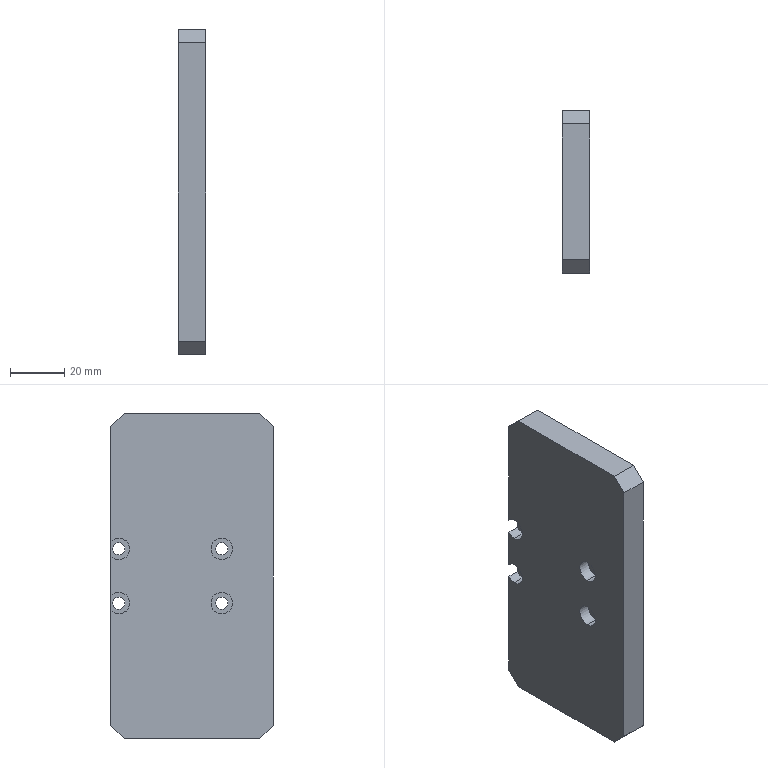Component | SolidWorks | MainRotatingPlate-1 | 1 solid | 32 faces | box 10.01 x 60 x 120 mm | volume 70291 mm3 | cylinder 18 | plane 14 | commonest cylinder face diameters 8 x10 4.5 x8
build123d program:
from build123d import *

# Parameters (mm, degrees)
SKETCH1_W                                       = 120
SKETCH1_H                                       = 60
BOSS_EXTRUDE1_DEPTH                             = 10
CHAMFER1_SIZE                                   = 5
M4_HEX_SOCKET_HEAD_CAP_SCREW_CBORE1_D           = 4.5
M4_HEX_SOCKET_HEAD_CAP_SCREW_CBORE1_DEPTH       = 12.4
M4_HEX_SOCKET_HEAD_CAP_SCREW_CBORE1_CBORE_D     = 8
M4_HEX_SOCKET_HEAD_CAP_SCREW_CBORE1_CBORE_DEPTH = 4.4
M4_HEX_SOCKET_HEAD_CAP_SCREW_CBORE1_TIP         = 1.352


with BuildPart() as part:
    # Sketch1 → Boss-Extrude1 (new body)
    with BuildSketch(Plane.XY):
        Rectangle(SKETCH1_W, SKETCH1_H)
    extrude(amount=BOSS_EXTRUDE1_DEPTH)

    # Chamfer1
    chamfer1_edges = [part.edges().sort_by_distance(p)[0] for p in [
        (-60, 30, 5),
        (60, 30, 5),
        (60, -30, 5),
        (-60, -30, 5),
    ]]
    chamfer(chamfer1_edges, length=CHAMFER1_SIZE)

    # M4 Hex Socket Head Cap Screw CBORE1
    with Locations(Plane.XY.offset(10)):
        with Locations((-10, 11), (10, 11), (-10, -27), (10, -27)):
            CounterBoreHole(M4_HEX_SOCKET_HEAD_CAP_SCREW_CBORE1_D / 2, M4_HEX_SOCKET_HEAD_CAP_SCREW_CBORE1_CBORE_D / 2, M4_HEX_SOCKET_HEAD_CAP_SCREW_CBORE1_CBORE_DEPTH, depth=M4_HEX_SOCKET_HEAD_CAP_SCREW_CBORE1_DEPTH)
            with Locations((0, 0, -(M4_HEX_SOCKET_HEAD_CAP_SCREW_CBORE1_DEPTH + M4_HEX_SOCKET_HEAD_CAP_SCREW_CBORE1_TIP / 2))):  # 118° drill point
                Cone(0, M4_HEX_SOCKET_HEAD_CAP_SCREW_CBORE1_D / 2, M4_HEX_SOCKET_HEAD_CAP_SCREW_CBORE1_TIP, mode=Mode.SUBTRACT)


solid = part.part

# Placed as in the assembly
solid = solid.moved(Location((1842.163, 3833.741, 1079.241), (180, -90, 0)))
STEP:
#1=COLOUR_RGB('',0.7922,0.8196,0.9333);
#2=FILL_AREA_STYLE_COLOUR('',#1);
#3=FILL_AREA_STYLE('',(#2));
#4=SURFACE_STYLE_FILL_AREA(#3);
#5=SURFACE_SIDE_STYLE('',(#4));
#6=SURFACE_STYLE_USAGE(.BOTH.,#5);
#7=PRESENTATION_STYLE_ASSIGNMENT((#6));
#8=CARTESIAN_POINT('',(72.306,150.502,43.041));
#9=VERTEX_POINT('',#8);
#10=CARTESIAN_POINT('',(72.306,150.502,42.726));
#11=VERTEX_POINT('',#10);
#12=CARTESIAN_POINT('',(72.306,150.502,42.884));
#13=DIRECTION('',(-1.,-0.0001552,-0.));
#14=DIRECTION('',(0.,0.,-1.));
#15=AXIS2_PLACEMENT_3D('',#12,#13,#14);
#16=CIRCLE('',#15,0.1575);
#17=EDGE_CURVE('',#9,#11,#16,.T.);
#18=ORIENTED_EDGE('',*,*,#17,.F.);
#19=CARTESIAN_POINT('',(72.132,150.502,43.041));
#20=VERTEX_POINT('',#19);
#21=CARTESIAN_POINT('',(72.132,150.502,43.041));
#22=DIRECTION('',(-1.,-0.0001552,-0.));
#23=VECTOR('',#22,39.37);
#24=LINE('',#21,#23);
#25=EDGE_CURVE('',#9,#20,#24,.T.);
#26=ORIENTED_EDGE('',*,*,#25,.T.);
#27=CARTESIAN_POINT('',(72.132,150.502,42.726));
#28=VERTEX_POINT('',#27);
#29=CARTESIAN_POINT('',(72.132,150.502,42.884));
#30=DIRECTION('',(-1.,-0.0001552,-0.));
#31=DIRECTION('',(0.,0.,-1.));
#32=AXIS2_PLACEMENT_3D('',#29,#30,#31);
#33=CIRCLE('',#32,0.1575);
#34=EDGE_CURVE('',#20,#28,#33,.T.);
#35=ORIENTED_EDGE('',*,*,#34,.T.);
#36=CARTESIAN_POINT('',(72.132,150.502,42.726));
#37=DIRECTION('',(-1.,-0.0001552,-0.));
#38=VECTOR('',#37,39.37);
#39=LINE('',#36,#38);
#40=EDGE_CURVE('',#11,#28,#39,.T.);
#41=ORIENTED_EDGE('',*,*,#40,.F.);
#42=EDGE_LOOP('',(#18,#26,#35,#41));
#43=FACE_OUTER_BOUND('',#42,.T.);
#44=CARTESIAN_POINT('',(72.132,150.502,42.884));
#45=DIRECTION('',(-1.,-0.0001552,-0.));
#46=DIRECTION('',(0.,0.,-1.));
#47=AXIS2_PLACEMENT_3D('',#44,#45,#46);
#48=CYLINDRICAL_SURFACE('',#47,0.1575);
#49=ADVANCED_FACE('',(#43),#48,.F.);
#50=CARTESIAN_POINT('',(72.526,150.502,42.972));
#51=VERTEX_POINT('',#50);
#52=CARTESIAN_POINT('',(72.526,150.502,42.795));
#53=VERTEX_POINT('',#52);
#54=CARTESIAN_POINT('',(72.526,150.502,42.884));
#55=DIRECTION('',(-1.,-0.0001552,-0.));
#56=DIRECTION('',(0.,0.,-1.));
#57=AXIS2_PLACEMENT_3D('',#54,#55,#56);
#58=CIRCLE('',#57,0.08858);
#59=EDGE_CURVE('',#51,#53,#58,.T.);
#60=ORIENTED_EDGE('',*,*,#59,.F.);
#61=CARTESIAN_POINT('',(72.306,150.502,42.972));
#62=VERTEX_POINT('',#61);
#63=CARTESIAN_POINT('',(72.132,150.502,42.972));
#64=DIRECTION('',(-1.,-0.0001552,-0.));
#65=VECTOR('',#64,39.37);
#66=LINE('',#63,#65);
#67=EDGE_CURVE('',#51,#62,#66,.T.);
#68=ORIENTED_EDGE('',*,*,#67,.T.);
#69=CARTESIAN_POINT('',(72.306,150.502,42.795));
#70=VERTEX_POINT('',#69);
#71=CARTESIAN_POINT('',(72.306,150.502,42.884));
#72=DIRECTION('',(-1.,-0.0001552,-0.));
#73=DIRECTION('',(0.,0.,-1.));
#74=AXIS2_PLACEMENT_3D('',#71,#72,#73);
#75=CIRCLE('',#74,0.08858);
#76=EDGE_CURVE('',#62,#70,#75,.T.);
#77=ORIENTED_EDGE('',*,*,#76,.T.);
#78=CARTESIAN_POINT('',(72.132,150.502,42.795));
#79=DIRECTION('',(-1.,-0.0001552,-0.));
#80=VECTOR('',#79,39.37);
#81=LINE('',#78,#80);
#82=EDGE_CURVE('',#53,#70,#81,.T.);
#83=ORIENTED_EDGE('',*,*,#82,.F.);
#84=EDGE_LOOP('',(#60,#68,#77,#83));
#85=FACE_OUTER_BOUND('',#84,.T.);
#86=CARTESIAN_POINT('',(72.132,150.502,42.884));
#87=DIRECTION('',(-1.,-0.0001552,-0.));
#88=DIRECTION('',(0.,0.,-1.));
#89=AXIS2_PLACEMENT_3D('',#86,#87,#88);
#90=CYLINDRICAL_SURFACE('',#89,0.08858);
#91=ADVANCED_FACE('',(#85),#90,.F.);
#92=CARTESIAN_POINT('',(72.306,150.502,42.254));
#93=VERTEX_POINT('',#92);
#94=CARTESIAN_POINT('',(72.306,150.502,41.939));
#95=VERTEX_POINT('',#94);
#96=CARTESIAN_POINT('',(72.306,150.502,42.096));
#97=DIRECTION('',(-1.,-0.0001552,-0.));
#98=DIRECTION('',(0.,0.,-1.));
#99=AXIS2_PLACEMENT_3D('',#96,#97,#98);
#100=CIRCLE('',#99,0.1575);
#101=EDGE_CURVE('',#93,#95,#100,.T.);
#102=ORIENTED_EDGE('',*,*,#101,.F.);
#103=CARTESIAN_POINT('',(72.132,150.502,42.254));
#104=VERTEX_POINT('',#103);
#105=CARTESIAN_POINT('',(72.132,150.502,42.254));
#106=DIRECTION('',(-1.,-0.0001552,-0.));
#107=VECTOR('',#106,39.37);
#108=LINE('',#105,#107);
#109=EDGE_CURVE('',#93,#104,#108,.T.);
#110=ORIENTED_EDGE('',*,*,#109,.T.);
#111=CARTESIAN_POINT('',(72.132,150.502,41.939));
#112=VERTEX_POINT('',#111);
#113=CARTESIAN_POINT('',(72.132,150.502,42.096));
#114=DIRECTION('',(-1.,-0.0001552,-0.));
#115=DIRECTION('',(0.,0.,-1.));
#116=AXIS2_PLACEMENT_3D('',#113,#114,#115);
#117=CIRCLE('',#116,0.1575);
#118=EDGE_CURVE('',#104,#112,#117,.T.);
#119=ORIENTED_EDGE('',*,*,#118,.T.);
#120=CARTESIAN_POINT('',(72.132,150.502,41.939));
#121=DIRECTION('',(-1.,-0.0001552,-0.));
#122=VECTOR('',#121,39.37);
#123=LINE('',#120,#122);
#124=EDGE_CURVE('',#95,#112,#123,.T.);
#125=ORIENTED_EDGE('',*,*,#124,.F.);
#126=EDGE_LOOP('',(#102,#110,#119,#125));
#127=FACE_OUTER_BOUND('',#126,.T.);
#128=CARTESIAN_POINT('',(72.132,150.502,42.096));
#129=DIRECTION('',(-1.,-0.0001552,-0.));
#130=DIRECTION('',(0.,0.,-1.));
#131=AXIS2_PLACEMENT_3D('',#128,#129,#130);
#132=CYLINDRICAL_SURFACE('',#131,0.1575);
#133=ADVANCED_FACE('',(#127),#132,.F.);
#134=CARTESIAN_POINT('',(72.526,150.502,42.185));
#135=VERTEX_POINT('',#134);
#136=CARTESIAN_POINT('',(72.526,150.502,42.008));
#137=VERTEX_POINT('',#136);
#138=CARTESIAN_POINT('',(72.526,150.502,42.096));
#139=DIRECTION('',(-1.,-0.0001552,-0.));
#140=DIRECTION('',(0.,0.,-1.));
#141=AXIS2_PLACEMENT_3D('',#138,#139,#140);
#142=CIRCLE('',#141,0.08858);
#143=EDGE_CURVE('',#135,#137,#142,.T.);
#144=ORIENTED_EDGE('',*,*,#143,.F.);
#145=CARTESIAN_POINT('',(72.306,150.502,42.185));
#146=VERTEX_POINT('',#145);
#147=CARTESIAN_POINT('',(72.132,150.502,42.185));
#148=DIRECTION('',(-1.,-0.0001552,-0.));
#149=VECTOR('',#148,39.37);
#150=LINE('',#147,#149);
#151=EDGE_CURVE('',#135,#146,#150,.T.);
#152=ORIENTED_EDGE('',*,*,#151,.T.);
#153=CARTESIAN_POINT('',(72.306,150.502,42.008));
#154=VERTEX_POINT('',#153);
#155=CARTESIAN_POINT('',(72.306,150.502,42.096));
#156=DIRECTION('',(-1.,-0.0001552,-0.));
#157=DIRECTION('',(0.,0.,-1.));
#158=AXIS2_PLACEMENT_3D('',#155,#156,#157);
#159=CIRCLE('',#158,0.08858);
#160=EDGE_CURVE('',#146,#154,#159,.T.);
#161=ORIENTED_EDGE('',*,*,#160,.T.);
#162=CARTESIAN_POINT('',(72.132,150.502,42.008));
#163=DIRECTION('',(-1.,-0.0001552,-0.));
#164=VECTOR('',#163,39.37);
#165=LINE('',#162,#164);
#166=EDGE_CURVE('',#137,#154,#165,.T.);
#167=ORIENTED_EDGE('',*,*,#166,.F.);
#168=EDGE_LOOP('',(#144,#152,#161,#167));
#169=FACE_OUTER_BOUND('',#168,.T.);
#170=CARTESIAN_POINT('',(72.132,150.502,42.096));
#171=DIRECTION('',(-1.,-0.0001552,-0.));
#172=DIRECTION('',(0.,0.,-1.));
#173=AXIS2_PLACEMENT_3D('',#170,#171,#172);
#174=CYLINDRICAL_SURFACE('',#173,0.08858);
#175=ADVANCED_FACE('',(#169),#174,.F.);
#176=CARTESIAN_POINT('',(72.526,151.998,42.972));
#177=VERTEX_POINT('',#176);
#178=CARTESIAN_POINT('',(72.526,151.998,42.795));
#179=VERTEX_POINT('',#178);
#180=CARTESIAN_POINT('',(72.526,151.998,42.884));
#181=DIRECTION('',(-1.,-0.0001552,-0.));
#182=DIRECTION('',(0.,0.,-1.));
#183=AXIS2_PLACEMENT_3D('',#180,#181,#182);
#184=CIRCLE('',#183,0.08858);
#185=EDGE_CURVE('',#177,#179,#184,.T.);
#186=ORIENTED_EDGE('',*,*,#185,.F.);
#187=CARTESIAN_POINT('',(72.305,151.998,42.972));
#188=VERTEX_POINT('',#187);
#189=CARTESIAN_POINT('',(72.132,151.998,42.972));
#190=DIRECTION('',(-1.,-0.0001552,-0.));
#191=VECTOR('',#190,39.37);
#192=LINE('',#189,#191);
#193=EDGE_CURVE('',#177,#188,#192,.T.);
#194=ORIENTED_EDGE('',*,*,#193,.T.);
#195=CARTESIAN_POINT('',(72.305,151.998,42.795));
#196=VERTEX_POINT('',#195);
#197=CARTESIAN_POINT('',(72.305,151.998,42.884));
#198=DIRECTION('',(-1.,-0.0001552,-0.));
#199=DIRECTION('',(0.,0.,-1.));
#200=AXIS2_PLACEMENT_3D('',#197,#198,#199);
#201=CIRCLE('',#200,0.08858);
#202=EDGE_CURVE('',#188,#196,#201,.T.);
#203=ORIENTED_EDGE('',*,*,#202,.T.);
#204=CARTESIAN_POINT('',(72.132,151.998,42.795));
#205=DIRECTION('',(-1.,-0.0001552,-0.));
#206=VECTOR('',#205,39.37);
#207=LINE('',#204,#206);
#208=EDGE_CURVE('',#179,#196,#207,.T.);
#209=ORIENTED_EDGE('',*,*,#208,.F.);
#210=EDGE_LOOP('',(#186,#194,#203,#209));
#211=FACE_OUTER_BOUND('',#210,.T.);
#212=CARTESIAN_POINT('',(72.132,151.998,42.884));
#213=DIRECTION('',(-1.,-0.0001552,-0.));
#214=DIRECTION('',(0.,0.,-1.));
#215=AXIS2_PLACEMENT_3D('',#212,#213,#214);
#216=CYLINDRICAL_SURFACE('',#215,0.08858);
#217=ADVANCED_FACE('',(#211),#216,.F.);
#218=CARTESIAN_POINT('',(72.305,151.998,43.041));
#219=VERTEX_POINT('',#218);
#220=CARTESIAN_POINT('',(72.305,152.116,42.988));
#221=VERTEX_POINT('',#220);
#222=CARTESIAN_POINT('',(72.305,151.998,42.884));
#223=DIRECTION('',(-1.,-0.0001552,-0.));
#224=DIRECTION('',(0.,0.,-1.));
#225=AXIS2_PLACEMENT_3D('',#222,#223,#224);
#226=CIRCLE('',#225,0.1575);
#227=EDGE_CURVE('',#219,#221,#226,.T.);
#228=ORIENTED_EDGE('',*,*,#227,.F.);
#229=CARTESIAN_POINT('',(72.132,151.998,43.041));
#230=VERTEX_POINT('',#229);
#231=CARTESIAN_POINT('',(72.132,151.998,43.041));
#232=DIRECTION('',(-1.,-0.0001552,-0.));
#233=VECTOR('',#232,39.37);
#234=LINE('',#231,#233);
#235=EDGE_CURVE('',#219,#230,#234,.T.);
#236=ORIENTED_EDGE('',*,*,#235,.T.);
#237=CARTESIAN_POINT('',(72.132,152.116,42.988));
#238=VERTEX_POINT('',#237);
#239=CARTESIAN_POINT('',(72.132,151.998,42.884));
#240=DIRECTION('',(-1.,-0.0001552,-0.));
#241=DIRECTION('',(0.,0.,-1.));
#242=AXIS2_PLACEMENT_3D('',#239,#240,#241);
#243=CIRCLE('',#242,0.1575);
#244=EDGE_CURVE('',#230,#238,#243,.T.);
#245=ORIENTED_EDGE('',*,*,#244,.T.);
#246=CARTESIAN_POINT('',(72.132,152.116,42.988));
#247=DIRECTION('',(-1.,-0.0001552,-0.));
#248=VECTOR('',#247,39.37);
#249=LINE('',#246,#248);
#250=EDGE_CURVE('',#221,#238,#249,.T.);
#251=ORIENTED_EDGE('',*,*,#250,.F.);
#252=EDGE_LOOP('',(#228,#236,#245,#251));
#253=FACE_OUTER_BOUND('',#252,.T.);
#254=CARTESIAN_POINT('',(72.132,151.998,42.884));
#255=DIRECTION('',(-1.,-0.0001552,-0.));
#256=DIRECTION('',(0.,0.,-1.));
#257=AXIS2_PLACEMENT_3D('',#254,#255,#256);
#258=CYLINDRICAL_SURFACE('',#257,0.1575);
#259=ADVANCED_FACE('',(#253),#258,.F.);
#260=ORIENTED_EDGE('',*,*,#235,.F.);
#261=CARTESIAN_POINT('',(72.305,151.998,42.726));
#262=VERTEX_POINT('',#261);
#263=CARTESIAN_POINT('',(72.305,151.998,42.884));
#264=DIRECTION('',(-1.,-0.0001552,-0.));
#265=DIRECTION('',(0.,0.,-1.));
#266=AXIS2_PLACEMENT_3D('',#263,#264,#265);
#267=CIRCLE('',#266,0.1575);
#268=EDGE_CURVE('',#262,#219,#267,.T.);
#269=ORIENTED_EDGE('',*,*,#268,.F.);
#270=CARTESIAN_POINT('',(72.132,151.998,42.726));
#271=VERTEX_POINT('',#270);
#272=CARTESIAN_POINT('',(72.132,151.998,42.726));
#273=DIRECTION('',(-1.,-0.0001552,-0.));
#274=VECTOR('',#273,39.37);
#275=LINE('',#272,#274);
#276=EDGE_CURVE('',#262,#271,#275,.T.);
#277=ORIENTED_EDGE('',*,*,#276,.T.);
#278=CARTESIAN_POINT('',(72.132,151.998,42.884));
#279=DIRECTION('',(-1.,-0.0001552,-0.));
#280=DIRECTION('',(0.,0.,-1.));
#281=AXIS2_PLACEMENT_3D('',#278,#279,#280);
#282=CIRCLE('',#281,0.1575);
#283=EDGE_CURVE('',#271,#230,#282,.T.);
#284=ORIENTED_EDGE('',*,*,#283,.T.);
#285=EDGE_LOOP('',(#260,#269,#277,#284));
#286=FACE_OUTER_BOUND('',#285,.T.);
#287=CARTESIAN_POINT('',(72.132,151.998,42.884));
#288=DIRECTION('',(-1.,-0.0001552,-0.));
#289=DIRECTION('',(0.,0.,-1.));
#290=AXIS2_PLACEMENT_3D('',#287,#288,#289);
#291=CYLINDRICAL_SURFACE('',#290,0.1575);
#292=ADVANCED_FACE('',(#286),#291,.F.);
#293=CARTESIAN_POINT('',(72.526,151.998,42.185));
#294=VERTEX_POINT('',#293);
#295=CARTESIAN_POINT('',(72.526,151.998,42.008));
#296=VERTEX_POINT('',#295);
#297=CARTESIAN_POINT('',(72.526,151.998,42.096));
#298=DIRECTION('',(-1.,-0.0001552,-0.));
#299=DIRECTION('',(0.,0.,-1.));
#300=AXIS2_PLACEMENT_3D('',#297,#298,#299);
#301=CIRCLE('',#300,0.08858);
#302=EDGE_CURVE('',#294,#296,#301,.T.);
#303=ORIENTED_EDGE('',*,*,#302,.F.);
#304=CARTESIAN_POINT('',(72.305,151.998,42.185));
#305=VERTEX_POINT('',#304);
#306=CARTESIAN_POINT('',(72.132,151.998,42.185));
#307=DIRECTION('',(-1.,-0.0001552,-0.));
#308=VECTOR('',#307,39.37);
#309=LINE('',#306,#308);
#310=EDGE_CURVE('',#294,#305,#309,.T.);
#311=ORIENTED_EDGE('',*,*,#310,.T.);
#312=CARTESIAN_POINT('',(72.305,151.998,42.008));
#313=VERTEX_POINT('',#312);
#314=CARTESIAN_POINT('',(72.305,151.998,42.096));
#315=DIRECTION('',(-1.,-0.0001552,-0.));
#316=DIRECTION('',(0.,0.,-1.));
#317=AXIS2_PLACEMENT_3D('',#314,#315,#316);
#318=CIRCLE('',#317,0.08858);
#319=EDGE_CURVE('',#305,#313,#318,.T.);
#320=ORIENTED_EDGE('',*,*,#319,.T.);
#321=CARTESIAN_POINT('',(72.132,151.998,42.008));
#322=DIRECTION('',(-1.,-0.0001552,-0.));
#323=VECTOR('',#322,39.37);
#324=LINE('',#321,#323);
#325=EDGE_CURVE('',#296,#313,#324,.T.);
#326=ORIENTED_EDGE('',*,*,#325,.F.);
#327=EDGE_LOOP('',(#303,#311,#320,#326));
#328=FACE_OUTER_BOUND('',#327,.T.);
#329=CARTESIAN_POINT('',(72.132,151.998,42.096));
#330=DIRECTION('',(-1.,-0.0001552,-0.));
#331=DIRECTION('',(0.,0.,-1.));
#332=AXIS2_PLACEMENT_3D('',#329,#330,#331);
#333=CYLINDRICAL_SURFACE('',#332,0.08858);
#334=ADVANCED_FACE('',(#328),#333,.F.);
#335=CARTESIAN_POINT('',(72.305,151.998,42.254));
#336=VERTEX_POINT('',#335);
#337=CARTESIAN_POINT('',(72.305,152.116,42.2));
#338=VERTEX_POINT('',#337);
#339=CARTESIAN_POINT('',(72.305,151.998,42.096));
#340=DIRECTION('',(-1.,-0.0001552,-0.));
#341=DIRECTION('',(0.,0.,-1.));
#342=AXIS2_PLACEMENT_3D('',#339,#340,#341);
#343=CIRCLE('',#342,0.1575);
#344=EDGE_CURVE('',#336,#338,#343,.T.);
#345=ORIENTED_EDGE('',*,*,#344,.F.);
#346=CARTESIAN_POINT('',(72.132,151.998,42.254));
#347=VERTEX_POINT('',#346);
#348=CARTESIAN_POINT('',(72.132,151.998,42.254));
#349=DIRECTION('',(-1.,-0.0001552,-0.));
#350=VECTOR('',#349,39.37);
#351=LINE('',#348,#350);
#352=EDGE_CURVE('',#336,#347,#351,.T.);
#353=ORIENTED_EDGE('',*,*,#352,.T.);
#354=CARTESIAN_POINT('',(72.132,152.116,42.2));
#355=VERTEX_POINT('',#354);
#356=CARTESIAN_POINT('',(72.132,151.998,42.096));
#357=DIRECTION('',(-1.,-0.0001552,-0.));
#358=DIRECTION('',(0.,0.,-1.));
#359=AXIS2_PLACEMENT_3D('',#356,#357,#358);
#360=CIRCLE('',#359,0.1575);
#361=EDGE_CURVE('',#347,#355,#360,.T.);
#362=ORIENTED_EDGE('',*,*,#361,.T.);
#363=CARTESIAN_POINT('',(72.132,152.116,42.2));
#364=DIRECTION('',(-1.,-0.0001552,-0.));
#365=VECTOR('',#364,39.37);
#366=LINE('',#363,#365);
#367=EDGE_CURVE('',#338,#355,#366,.T.);
#368=ORIENTED_EDGE('',*,*,#367,.F.);
#369=EDGE_LOOP('',(#345,#353,#362,#368));
#370=FACE_OUTER_BOUND('',#369,.T.);
#371=CARTESIAN_POINT('',(72.132,151.998,42.096));
#372=DIRECTION('',(-1.,-0.0001552,-0.));
#373=DIRECTION('',(0.,0.,-1.));
#374=AXIS2_PLACEMENT_3D('',#371,#372,#373);
#375=CYLINDRICAL_SURFACE('',#374,0.1575);
#376=ADVANCED_FACE('',(#370),#375,.F.);
#377=ORIENTED_EDGE('',*,*,#352,.F.);
#378=CARTESIAN_POINT('',(72.305,151.998,41.939));
#379=VERTEX_POINT('',#378);
#380=CARTESIAN_POINT('',(72.305,151.998,42.096));
#381=DIRECTION('',(-1.,-0.0001552,-0.));
#382=DIRECTION('',(0.,0.,-1.));
#383=AXIS2_PLACEMENT_3D('',#380,#381,#382);
#384=CIRCLE('',#383,0.1575);
#385=EDGE_CURVE('',#379,#336,#384,.T.);
#386=ORIENTED_EDGE('',*,*,#385,.F.);
#387=CARTESIAN_POINT('',(72.132,151.998,41.939));
#388=VERTEX_POINT('',#387);
#389=CARTESIAN_POINT('',(72.132,151.998,41.939));
#390=DIRECTION('',(-1.,-0.0001552,-0.));
#391=VECTOR('',#390,39.37);
#392=LINE('',#389,#391);
#393=EDGE_CURVE('',#379,#388,#392,.T.);
#394=ORIENTED_EDGE('',*,*,#393,.T.);
#395=CARTESIAN_POINT('',(72.132,151.998,42.096));
#396=DIRECTION('',(-1.,-0.0001552,-0.));
#397=DIRECTION('',(0.,0.,-1.));
#398=AXIS2_PLACEMENT_3D('',#395,#396,#397);
#399=CIRCLE('',#398,0.1575);
#400=EDGE_CURVE('',#388,#347,#399,.T.);
#401=ORIENTED_EDGE('',*,*,#400,.T.);
#402=EDGE_LOOP('',(#377,#386,#394,#401));
#403=FACE_OUTER_BOUND('',#402,.T.);
#404=CARTESIAN_POINT('',(72.132,151.998,42.096));
#405=DIRECTION('',(-1.,-0.0001552,-0.));
#406=DIRECTION('',(0.,0.,-1.));
#407=AXIS2_PLACEMENT_3D('',#404,#405,#406);
#408=CYLINDRICAL_SURFACE('',#407,0.1575);
#409=ADVANCED_FACE('',(#403),#408,.F.);
#410=CARTESIAN_POINT('',(72.526,149.95,44.852));
#411=VERTEX_POINT('',#410);
#412=CARTESIAN_POINT('',(72.526,151.919,44.852));
#413=VERTEX_POINT('',#412);
#414=CARTESIAN_POINT('',(72.526,152.116,44.852));
#415=DIRECTION('',(-0.0001552,1.,0.));
#416=VECTOR('',#415,39.37);
#417=LINE('',#414,#416);
#418=EDGE_CURVE('',#411,#413,#417,.T.);
#419=ORIENTED_EDGE('',*,*,#418,.T.);
#420=CARTESIAN_POINT('',(72.132,151.919,44.852));
#421=VERTEX_POINT('',#420);
#422=CARTESIAN_POINT('',(72.132,151.919,44.852));
#423=DIRECTION('',(-1.,-0.0001552,-0.));
#424=VECTOR('',#423,39.37);
#425=LINE('',#422,#424);
#426=EDGE_CURVE('',#413,#421,#425,.T.);
#427=ORIENTED_EDGE('',*,*,#426,.T.);
#428=CARTESIAN_POINT('',(72.133,149.95,44.852));
#429=VERTEX_POINT('',#428);
#430=CARTESIAN_POINT('',(72.132,152.116,44.852));
#431=DIRECTION('',(-0.0001552,1.,0.));
#432=VECTOR('',#431,39.37);
#433=LINE('',#430,#432);
#434=EDGE_CURVE('',#429,#421,#433,.T.);
#435=ORIENTED_EDGE('',*,*,#434,.F.);
#436=CARTESIAN_POINT('',(72.133,149.95,44.852));
#437=DIRECTION('',(1.,0.0001552,0.));
#438=VECTOR('',#437,39.37);
#439=LINE('',#436,#438);
#440=EDGE_CURVE('',#429,#411,#439,.T.);
#441=ORIENTED_EDGE('',*,*,#440,.T.);
#442=EDGE_LOOP('',(#419,#427,#435,#441));
#443=FACE_OUTER_BOUND('',#442,.T.);
#444=CARTESIAN_POINT('',(72.132,152.116,44.852));
#445=DIRECTION('',(0.,0.,-1.));
#446=DIRECTION('',(1.,0.0001552,0.));
#447=AXIS2_PLACEMENT_3D('',#444,#445,#446);
#448=PLANE('',#447);
#449=ADVANCED_FACE('',(#443),#448,.F.);
#450=CARTESIAN_POINT('',(72.305,152.116,42.779));
#451=VERTEX_POINT('',#450);
#452=CARTESIAN_POINT('',(72.305,152.116,40.128));
#453=DIRECTION('',(-0.,0.,1.));
#454=VECTOR('',#453,39.37);
#455=LINE('',#452,#454);
#456=EDGE_CURVE('',#451,#221,#455,.T.);
#457=ORIENTED_EDGE('',*,*,#456,.T.);
#458=ORIENTED_EDGE('',*,*,#250,.T.);
#459=CARTESIAN_POINT('',(72.132,152.116,44.655));
#460=VERTEX_POINT('',#459);
#461=CARTESIAN_POINT('',(72.132,152.116,40.128));
#462=DIRECTION('',(0.,-0.,-1.));
#463=VECTOR('',#462,39.37);
#464=LINE('',#461,#463);
#465=EDGE_CURVE('',#460,#238,#464,.T.);
#466=ORIENTED_EDGE('',*,*,#465,.F.);
#467=CARTESIAN_POINT('',(72.526,152.116,44.655));
#468=VERTEX_POINT('',#467);
#469=CARTESIAN_POINT('',(72.132,152.116,44.655));
#470=DIRECTION('',(1.,0.0001552,0.));
#471=VECTOR('',#470,39.37);
#472=LINE('',#469,#471);
#473=EDGE_CURVE('',#460,#468,#472,.T.);
#474=ORIENTED_EDGE('',*,*,#473,.T.);
#475=CARTESIAN_POINT('',(72.526,152.116,40.324));
#476=VERTEX_POINT('',#475);
#477=CARTESIAN_POINT('',(72.526,152.116,40.128));
#478=DIRECTION('',(0.,-0.,-1.));
#479=VECTOR('',#478,39.37);
#480=LINE('',#477,#479);
#481=EDGE_CURVE('',#468,#476,#480,.T.);
#482=ORIENTED_EDGE('',*,*,#481,.T.);
#483=CARTESIAN_POINT('',(72.132,152.116,40.324));
#484=VERTEX_POINT('',#483);
#485=CARTESIAN_POINT('',(72.132,152.116,40.324));
#486=DIRECTION('',(-1.,-0.0001552,-0.));
#487=VECTOR('',#486,39.37);
#488=LINE('',#485,#487);
#489=EDGE_CURVE('',#476,#484,#488,.T.);
#490=ORIENTED_EDGE('',*,*,#489,.T.);
#491=CARTESIAN_POINT('',(72.132,152.116,41.992));
#492=VERTEX_POINT('',#491);
#493=CARTESIAN_POINT('',(72.132,152.116,40.128));
#494=DIRECTION('',(0.,-0.,-1.));
#495=VECTOR('',#494,39.37);
#496=LINE('',#493,#495);
#497=EDGE_CURVE('',#492,#484,#496,.T.);
#498=ORIENTED_EDGE('',*,*,#497,.F.);
#499=CARTESIAN_POINT('',(72.305,152.116,41.992));
#500=VERTEX_POINT('',#499);
#501=CARTESIAN_POINT('',(72.132,152.116,41.992));
#502=DIRECTION('',(1.,0.0001552,0.));
#503=VECTOR('',#502,39.37);
#504=LINE('',#501,#503);
#505=EDGE_CURVE('',#492,#500,#504,.T.);
#506=ORIENTED_EDGE('',*,*,#505,.T.);
#507=CARTESIAN_POINT('',(72.305,152.116,40.128));
#508=DIRECTION('',(-0.,0.,1.));
#509=VECTOR('',#508,39.37);
#510=LINE('',#507,#509);
#511=EDGE_CURVE('',#500,#338,#510,.T.);
#512=ORIENTED_EDGE('',*,*,#511,.T.);
#513=ORIENTED_EDGE('',*,*,#367,.T.);
#514=CARTESIAN_POINT('',(72.132,152.116,42.779));
#515=VERTEX_POINT('',#514);
#516=CARTESIAN_POINT('',(72.132,152.116,40.128));
#517=DIRECTION('',(0.,-0.,-1.));
#518=VECTOR('',#517,39.37);
#519=LINE('',#516,#518);
#520=EDGE_CURVE('',#515,#355,#519,.T.);
#521=ORIENTED_EDGE('',*,*,#520,.F.);
#522=CARTESIAN_POINT('',(72.132,152.116,42.779));
#523=DIRECTION('',(1.,0.0001552,0.));
#524=VECTOR('',#523,39.37);
#525=LINE('',#522,#524);
#526=EDGE_CURVE('',#515,#451,#525,.T.);
#527=ORIENTED_EDGE('',*,*,#526,.T.);
#528=EDGE_LOOP('',(#457,#458,#466,#474,#482,#490,#498,#506,#512,#513,#521,#527));
#529=FACE_OUTER_BOUND('',#528,.T.);
#530=CARTESIAN_POINT('',(72.132,152.116,40.128));
#531=DIRECTION('',(0.0001552,-1.,0.));
#532=DIRECTION('',(-0.,0.,1.));
#533=AXIS2_PLACEMENT_3D('',#530,#531,#532);
#534=PLANE('',#533);
#535=ADVANCED_FACE('',(#529),#534,.F.);
#536=CARTESIAN_POINT('',(72.526,151.919,40.128));
#537=VERTEX_POINT('',#536);
#538=CARTESIAN_POINT('',(72.526,149.95,40.128));
#539=VERTEX_POINT('',#538);
#540=CARTESIAN_POINT('',(72.526,152.116,40.128));
#541=DIRECTION('',(0.0001552,-1.,-0.));
#542=VECTOR('',#541,39.37);
#543=LINE('',#540,#542);
#544=EDGE_CURVE('',#537,#539,#543,.T.);
#545=ORIENTED_EDGE('',*,*,#544,.T.);
#546=CARTESIAN_POINT('',(72.133,149.95,40.128));
#547=VERTEX_POINT('',#546);
#548=CARTESIAN_POINT('',(72.133,149.95,40.128));
#549=DIRECTION('',(-1.,-0.0001552,-0.));
#550=VECTOR('',#549,39.37);
#551=LINE('',#548,#550);
#552=EDGE_CURVE('',#539,#547,#551,.T.);
#553=ORIENTED_EDGE('',*,*,#552,.T.);
#554=CARTESIAN_POINT('',(72.132,151.919,40.128));
#555=VERTEX_POINT('',#554);
#556=CARTESIAN_POINT('',(72.132,152.116,40.128));
#557=DIRECTION('',(0.0001552,-1.,-0.));
#558=VECTOR('',#557,39.37);
#559=LINE('',#556,#558);
#560=EDGE_CURVE('',#555,#547,#559,.T.);
#561=ORIENTED_EDGE('',*,*,#560,.F.);
#562=CARTESIAN_POINT('',(72.132,151.919,40.128));
#563=DIRECTION('',(1.,0.0001552,0.));
#564=VECTOR('',#563,39.37);
#565=LINE('',#562,#564);
#566=EDGE_CURVE('',#555,#537,#565,.T.);
#567=ORIENTED_EDGE('',*,*,#566,.T.);
#568=EDGE_LOOP('',(#545,#553,#561,#567));
#569=FACE_OUTER_BOUND('',#568,.T.);
#570=CARTESIAN_POINT('',(72.132,152.116,40.128));
#571=DIRECTION('',(-0.,-0.,1.));
#572=DIRECTION('',(-1.,-0.0001552,-0.));
#573=AXIS2_PLACEMENT_3D('',#570,#571,#572);
#574=PLANE('',#573);
#575=ADVANCED_FACE('',(#569),#574,.F.);
#576=CARTESIAN_POINT('',(72.133,149.754,40.324));
#577=VERTEX_POINT('',#576);
#578=CARTESIAN_POINT('',(72.133,149.754,44.655));
#579=VERTEX_POINT('',#578);
#580=CARTESIAN_POINT('',(72.133,149.754,40.128));
#581=DIRECTION('',(-0.,0.,1.));
#582=VECTOR('',#581,39.37);
#583=LINE('',#580,#582);
#584=EDGE_CURVE('',#577,#579,#583,.T.);
#585=ORIENTED_EDGE('',*,*,#584,.F.);
#586=CARTESIAN_POINT('',(72.526,149.754,40.324));
#587=VERTEX_POINT('',#586);
#588=CARTESIAN_POINT('',(72.133,149.754,40.324));
#589=DIRECTION('',(1.,0.0001552,0.));
#590=VECTOR('',#589,39.37);
#591=LINE('',#588,#590);
#592=EDGE_CURVE('',#577,#587,#591,.T.);
#593=ORIENTED_EDGE('',*,*,#592,.T.);
#594=CARTESIAN_POINT('',(72.526,149.754,44.655));
#595=VERTEX_POINT('',#594);
#596=CARTESIAN_POINT('',(72.526,149.754,40.128));
#597=DIRECTION('',(-0.,0.,1.));
#598=VECTOR('',#597,39.37);
#599=LINE('',#596,#598);
#600=EDGE_CURVE('',#587,#595,#599,.T.);
#601=ORIENTED_EDGE('',*,*,#600,.T.);
#602=CARTESIAN_POINT('',(72.133,149.754,44.655));
#603=DIRECTION('',(-1.,-0.0001552,-0.));
#604=VECTOR('',#603,39.37);
#605=LINE('',#602,#604);
#606=EDGE_CURVE('',#595,#579,#605,.T.);
#607=ORIENTED_EDGE('',*,*,#606,.T.);
#608=EDGE_LOOP('',(#585,#593,#601,#607));
#609=FACE_OUTER_BOUND('',#608,.T.);
#610=CARTESIAN_POINT('',(72.133,149.754,40.128));
#611=DIRECTION('',(-0.0001552,1.,-0.));
#612=DIRECTION('',(0.,-0.,-1.));
#613=AXIS2_PLACEMENT_3D('',#610,#611,#612);
#614=PLANE('',#613);
#615=ADVANCED_FACE('',(#609),#614,.F.);
#616=CARTESIAN_POINT('',(72.132,150.502,42.884));
#617=DIRECTION('',(-1.,-0.0001552,-0.));
#618=DIRECTION('',(0.,0.,-1.));
#619=AXIS2_PLACEMENT_3D('',#616,#617,#618);
#620=CIRCLE('',#619,0.1575);
#621=EDGE_CURVE('',#28,#20,#620,.T.);
#622=ORIENTED_EDGE('',*,*,#621,.F.);
#623=ORIENTED_EDGE('',*,*,#34,.F.);
#624=EDGE_LOOP('',(#622,#623));
#625=FACE_BOUND('',#624,.T.);
#626=CARTESIAN_POINT('',(72.132,150.502,42.096));
#627=DIRECTION('',(-1.,-0.0001552,-0.));
#628=DIRECTION('',(0.,0.,-1.));
#629=AXIS2_PLACEMENT_3D('',#626,#627,#628);
#630=CIRCLE('',#629,0.1575);
#631=EDGE_CURVE('',#112,#104,#630,.T.);
#632=ORIENTED_EDGE('',*,*,#631,.F.);
#633=ORIENTED_EDGE('',*,*,#118,.F.);
#634=EDGE_LOOP('',(#632,#633));
#635=FACE_BOUND('',#634,.T.);
#636=CARTESIAN_POINT('',(72.132,151.998,42.884));
#637=DIRECTION('',(-1.,-0.0001552,-0.));
#638=DIRECTION('',(0.,0.,-1.));
#639=AXIS2_PLACEMENT_3D('',#636,#637,#638);
#640=CIRCLE('',#639,0.1575);
#641=EDGE_CURVE('',#515,#271,#640,.T.);
#642=ORIENTED_EDGE('',*,*,#641,.F.);
#643=ORIENTED_EDGE('',*,*,#520,.T.);
#644=ORIENTED_EDGE('',*,*,#361,.F.);
#645=ORIENTED_EDGE('',*,*,#400,.F.);
#646=CARTESIAN_POINT('',(72.132,151.998,42.096));
#647=DIRECTION('',(-1.,-0.0001552,-0.));
#648=DIRECTION('',(0.,0.,-1.));
#649=AXIS2_PLACEMENT_3D('',#646,#647,#648);
#650=CIRCLE('',#649,0.1575);
#651=EDGE_CURVE('',#492,#388,#650,.T.);
#652=ORIENTED_EDGE('',*,*,#651,.F.);
#653=ORIENTED_EDGE('',*,*,#497,.T.);
#654=CARTESIAN_POINT('',(72.132,152.608,40.817));
#655=DIRECTION('',(0.0001098,-0.7071,-0.7071));
#656=VECTOR('',#655,39.37);
#657=LINE('',#654,#656);
#658=EDGE_CURVE('',#484,#555,#657,.T.);
#659=ORIENTED_EDGE('',*,*,#658,.T.);
#660=ORIENTED_EDGE('',*,*,#560,.T.);
#661=CARTESIAN_POINT('',(72.133,149.261,40.817));
#662=DIRECTION('',(0.0001098,-0.7071,0.7071));
#663=VECTOR('',#662,39.37);
#664=LINE('',#661,#663);
#665=EDGE_CURVE('',#547,#577,#664,.T.);
#666=ORIENTED_EDGE('',*,*,#665,.T.);
#667=ORIENTED_EDGE('',*,*,#584,.T.);
#668=CARTESIAN_POINT('',(72.133,149.261,44.163));
#669=DIRECTION('',(-0.0001098,0.7071,0.7071));
#670=VECTOR('',#669,39.37);
#671=LINE('',#668,#670);
#672=EDGE_CURVE('',#579,#429,#671,.T.);
#673=ORIENTED_EDGE('',*,*,#672,.T.);
#674=ORIENTED_EDGE('',*,*,#434,.T.);
#675=CARTESIAN_POINT('',(72.132,152.608,44.163));
#676=DIRECTION('',(-0.0001098,0.7071,-0.7071));
#677=VECTOR('',#676,39.37);
#678=LINE('',#675,#677);
#679=EDGE_CURVE('',#421,#460,#678,.T.);
#680=ORIENTED_EDGE('',*,*,#679,.T.);
#681=ORIENTED_EDGE('',*,*,#465,.T.);
#682=ORIENTED_EDGE('',*,*,#244,.F.);
#683=ORIENTED_EDGE('',*,*,#283,.F.);
#684=EDGE_LOOP('',(#642,#643,#644,#645,#652,#653,#659,#660,#666,#667,#673,#674,#680,#681,#682,#683));
#685=FACE_OUTER_BOUND('',#684,.T.);
#686=CARTESIAN_POINT('',(72.132,150.935,42.49));
#687=DIRECTION('',(-1.,-0.0001552,-0.));
#688=DIRECTION('',(0.,0.,-1.));
#689=AXIS2_PLACEMENT_3D('',#686,#687,#688);
#690=PLANE('',#689);
#691=ADVANCED_FACE('',(#625,#635,#685),#690,.T.);
#692=CARTESIAN_POINT('',(72.526,150.502,42.884));
#693=DIRECTION('',(-1.,-0.0001552,-0.));
#694=DIRECTION('',(0.,0.,-1.));
#695=AXIS2_PLACEMENT_3D('',#692,#693,#694);
#696=CIRCLE('',#695,0.08858);
#697=EDGE_CURVE('',#53,#51,#696,.T.);
#698=ORIENTED_EDGE('',*,*,#697,.T.);
#699=ORIENTED_EDGE('',*,*,#59,.T.);
#700=EDGE_LOOP('',(#698,#699));
#701=FACE_BOUND('',#700,.T.);
#702=CARTESIAN_POINT('',(72.526,150.502,42.096));
#703=DIRECTION('',(-1.,-0.0001552,-0.));
#704=DIRECTION('',(0.,0.,-1.));
#705=AXIS2_PLACEMENT_3D('',#702,#703,#704);
#706=CIRCLE('',#705,0.08858);
#707=EDGE_CURVE('',#137,#135,#706,.T.);
#708=ORIENTED_EDGE('',*,*,#707,.T.);
#709=ORIENTED_EDGE('',*,*,#143,.T.);
#710=EDGE_LOOP('',(#708,#709));
#711=FACE_BOUND('',#710,.T.);
#712=CARTESIAN_POINT('',(72.526,151.998,42.884));
#713=DIRECTION('',(-1.,-0.0001552,-0.));
#714=DIRECTION('',(0.,0.,-1.));
#715=AXIS2_PLACEMENT_3D('',#712,#713,#714);
#716=CIRCLE('',#715,0.08858);
#717=EDGE_CURVE('',#179,#177,#716,.T.);
#718=ORIENTED_EDGE('',*,*,#717,.T.);
#719=ORIENTED_EDGE('',*,*,#185,.T.);
#720=EDGE_LOOP('',(#718,#719));
#721=FACE_BOUND('',#720,.T.);
#722=CARTESIAN_POINT('',(72.526,151.998,42.096));
#723=DIRECTION('',(-1.,-0.0001552,-0.));
#724=DIRECTION('',(0.,0.,-1.));
#725=AXIS2_PLACEMENT_3D('',#722,#723,#724);
#726=CIRCLE('',#725,0.08858);
#727=EDGE_CURVE('',#296,#294,#726,.T.);
#728=ORIENTED_EDGE('',*,*,#727,.T.);
#729=ORIENTED_EDGE('',*,*,#302,.T.);
#730=EDGE_LOOP('',(#728,#729));
#731=FACE_BOUND('',#730,.T.);
#732=ORIENTED_EDGE('',*,*,#600,.F.);
#733=CARTESIAN_POINT('',(72.526,149.754,40.324));
#734=DIRECTION('',(-0.0001098,0.7071,-0.7071));
#735=VECTOR('',#734,39.37);
#736=LINE('',#733,#735);
#737=EDGE_CURVE('',#587,#539,#736,.T.);
#738=ORIENTED_EDGE('',*,*,#737,.T.);
#739=ORIENTED_EDGE('',*,*,#544,.F.);
#740=CARTESIAN_POINT('',(72.526,151.919,40.128));
#741=DIRECTION('',(-0.0001098,0.7071,0.7071));
#742=VECTOR('',#741,39.37);
#743=LINE('',#740,#742);
#744=EDGE_CURVE('',#537,#476,#743,.T.);
#745=ORIENTED_EDGE('',*,*,#744,.T.);
#746=ORIENTED_EDGE('',*,*,#481,.F.);
#747=CARTESIAN_POINT('',(72.526,152.116,44.655));
#748=DIRECTION('',(0.0001098,-0.7071,0.7071));
#749=VECTOR('',#748,39.37);
#750=LINE('',#747,#749);
#751=EDGE_CURVE('',#468,#413,#750,.T.);
#752=ORIENTED_EDGE('',*,*,#751,.T.);
#753=ORIENTED_EDGE('',*,*,#418,.F.);
#754=CARTESIAN_POINT('',(72.526,149.95,44.852));
#755=DIRECTION('',(0.0001098,-0.7071,-0.7071));
#756=VECTOR('',#755,39.37);
#757=LINE('',#754,#756);
#758=EDGE_CURVE('',#411,#595,#757,.T.);
#759=ORIENTED_EDGE('',*,*,#758,.T.);
#760=EDGE_LOOP('',(#732,#738,#739,#745,#746,#752,#753,#759));
#761=FACE_OUTER_BOUND('',#760,.T.);
#762=CARTESIAN_POINT('',(72.526,150.935,42.49));
#763=DIRECTION('',(-1.,-0.0001552,-0.));
#764=DIRECTION('',(0.,0.,-1.));
#765=AXIS2_PLACEMENT_3D('',#762,#763,#764);
#766=PLANE('',#765);
#767=ADVANCED_FACE('',(#701,#711,#721,#731,#761),#766,.F.);
#768=ORIENTED_EDGE('',*,*,#665,.F.);
#769=ORIENTED_EDGE('',*,*,#552,.F.);
#770=ORIENTED_EDGE('',*,*,#737,.F.);
#771=ORIENTED_EDGE('',*,*,#592,.F.);
#772=EDGE_LOOP('',(#768,#769,#770,#771));
#773=FACE_OUTER_BOUND('',#772,.T.);
#774=CARTESIAN_POINT('',(72.133,149.754,40.324));
#775=DIRECTION('',(-0.0001098,0.7071,0.7071));
#776=DIRECTION('',(1.,0.0001552,0.));
#777=AXIS2_PLACEMENT_3D('',#774,#775,#776);
#778=PLANE('',#777);
#779=ADVANCED_FACE('',(#773),#778,.F.);
#780=ORIENTED_EDGE('',*,*,#658,.F.);
#781=ORIENTED_EDGE('',*,*,#489,.F.);
#782=ORIENTED_EDGE('',*,*,#744,.F.);
#783=ORIENTED_EDGE('',*,*,#566,.F.);
#784=EDGE_LOOP('',(#780,#781,#782,#783));
#785=FACE_OUTER_BOUND('',#784,.T.);
#786=CARTESIAN_POINT('',(72.132,151.919,40.128));
#787=DIRECTION('',(0.0001098,-0.7071,0.7071));
#788=DIRECTION('',(1.,0.0001552,0.));
#789=AXIS2_PLACEMENT_3D('',#786,#787,#788);
#790=PLANE('',#789);
#791=ADVANCED_FACE('',(#785),#790,.F.);
#792=ORIENTED_EDGE('',*,*,#679,.F.);
#793=ORIENTED_EDGE('',*,*,#426,.F.);
#794=ORIENTED_EDGE('',*,*,#751,.F.);
#795=ORIENTED_EDGE('',*,*,#473,.F.);
#796=EDGE_LOOP('',(#792,#793,#794,#795));
#797=FACE_OUTER_BOUND('',#796,.T.);
#798=CARTESIAN_POINT('',(72.132,152.116,44.655));
#799=DIRECTION('',(0.0001098,-0.7071,-0.7071));
#800=DIRECTION('',(1.,0.0001552,0.));
#801=AXIS2_PLACEMENT_3D('',#798,#799,#800);
#802=PLANE('',#801);
#803=ADVANCED_FACE('',(#797),#802,.F.);
#804=ORIENTED_EDGE('',*,*,#672,.F.);
#805=ORIENTED_EDGE('',*,*,#606,.F.);
#806=ORIENTED_EDGE('',*,*,#758,.F.);
#807=ORIENTED_EDGE('',*,*,#440,.F.);
#808=EDGE_LOOP('',(#804,#805,#806,#807));
#809=FACE_OUTER_BOUND('',#808,.T.);
#810=CARTESIAN_POINT('',(72.133,149.95,44.852));
#811=DIRECTION('',(-0.0001098,0.7071,-0.7071));
#812=DIRECTION('',(1.,0.0001552,0.));
#813=AXIS2_PLACEMENT_3D('',#810,#811,#812);
#814=PLANE('',#813);
#815=ADVANCED_FACE('',(#809),#814,.F.);
#816=CARTESIAN_POINT('',(72.305,151.998,42.096));
#817=DIRECTION('',(-1.,-0.0001552,-0.));
#818=DIRECTION('',(0.,0.,-1.));
#819=AXIS2_PLACEMENT_3D('',#816,#817,#818);
#820=CIRCLE('',#819,0.08858);
#821=EDGE_CURVE('',#313,#305,#820,.T.);
#822=ORIENTED_EDGE('',*,*,#821,.F.);
#823=ORIENTED_EDGE('',*,*,#319,.F.);
#824=EDGE_LOOP('',(#822,#823));
#825=FACE_BOUND('',#824,.T.);
#826=CARTESIAN_POINT('',(72.305,151.998,42.096));
#827=DIRECTION('',(-1.,-0.0001552,-0.));
#828=DIRECTION('',(0.,0.,-1.));
#829=AXIS2_PLACEMENT_3D('',#826,#827,#828);
#830=CIRCLE('',#829,0.1575);
#831=EDGE_CURVE('',#500,#379,#830,.T.);
#832=ORIENTED_EDGE('',*,*,#831,.T.);
#833=ORIENTED_EDGE('',*,*,#385,.T.);
#834=ORIENTED_EDGE('',*,*,#344,.T.);
#835=ORIENTED_EDGE('',*,*,#511,.F.);
#836=EDGE_LOOP('',(#832,#833,#834,#835));
#837=FACE_OUTER_BOUND('',#836,.T.);
#838=CARTESIAN_POINT('',(72.305,151.998,42.008));
#839=DIRECTION('',(1.,0.0001552,0.));
#840=DIRECTION('',(-0.,-0.,1.));
#841=AXIS2_PLACEMENT_3D('',#838,#839,#840);
#842=PLANE('',#841);
#843=ADVANCED_FACE('',(#825,#837),#842,.F.);
#844=ORIENTED_EDGE('',*,*,#393,.F.);
#845=ORIENTED_EDGE('',*,*,#831,.F.);
#846=ORIENTED_EDGE('',*,*,#505,.F.);
#847=ORIENTED_EDGE('',*,*,#651,.T.);
#848=EDGE_LOOP('',(#844,#845,#846,#847));
#849=FACE_OUTER_BOUND('',#848,.T.);
#850=CARTESIAN_POINT('',(72.132,151.998,42.096));
#851=DIRECTION('',(-1.,-0.0001552,-0.));
#852=DIRECTION('',(0.,0.,-1.));
#853=AXIS2_PLACEMENT_3D('',#850,#851,#852);
#854=CYLINDRICAL_SURFACE('',#853,0.1575);
#855=ADVANCED_FACE('',(#849),#854,.F.);
#856=ORIENTED_EDGE('',*,*,#310,.F.);
#857=ORIENTED_EDGE('',*,*,#727,.F.);
#858=ORIENTED_EDGE('',*,*,#325,.T.);
#859=ORIENTED_EDGE('',*,*,#821,.T.);
#860=EDGE_LOOP('',(#856,#857,#858,#859));
#861=FACE_OUTER_BOUND('',#860,.T.);
#862=CARTESIAN_POINT('',(72.132,151.998,42.096));
#863=DIRECTION('',(-1.,-0.0001552,-0.));
#864=DIRECTION('',(0.,0.,-1.));
#865=AXIS2_PLACEMENT_3D('',#862,#863,#864);
#866=CYLINDRICAL_SURFACE('',#865,0.08858);
#867=ADVANCED_FACE('',(#861),#866,.F.);
#868=CARTESIAN_POINT('',(72.305,151.998,42.884));
#869=DIRECTION('',(-1.,-0.0001552,-0.));
#870=DIRECTION('',(0.,0.,-1.));
#871=AXIS2_PLACEMENT_3D('',#868,#869,#870);
#872=CIRCLE('',#871,0.08858);
#873=EDGE_CURVE('',#196,#188,#872,.T.);
#874=ORIENTED_EDGE('',*,*,#873,.F.);
#875=ORIENTED_EDGE('',*,*,#202,.F.);
#876=EDGE_LOOP('',(#874,#875));
#877=FACE_BOUND('',#876,.T.);
#878=CARTESIAN_POINT('',(72.305,151.998,42.884));
#879=DIRECTION('',(-1.,-0.0001552,-0.));
#880=DIRECTION('',(0.,0.,-1.));
#881=AXIS2_PLACEMENT_3D('',#878,#879,#880);
#882=CIRCLE('',#881,0.1575);
#883=EDGE_CURVE('',#451,#262,#882,.T.);
#884=ORIENTED_EDGE('',*,*,#883,.T.);
#885=ORIENTED_EDGE('',*,*,#268,.T.);
#886=ORIENTED_EDGE('',*,*,#227,.T.);
#887=ORIENTED_EDGE('',*,*,#456,.F.);
#888=EDGE_LOOP('',(#884,#885,#886,#887));
#889=FACE_OUTER_BOUND('',#888,.T.);
#890=CARTESIAN_POINT('',(72.305,151.998,42.795));
#891=DIRECTION('',(1.,0.0001552,0.));
#892=DIRECTION('',(-0.,-0.,1.));
#893=AXIS2_PLACEMENT_3D('',#890,#891,#892);
#894=PLANE('',#893);
#895=ADVANCED_FACE('',(#877,#889),#894,.F.);
#896=ORIENTED_EDGE('',*,*,#276,.F.);
#897=ORIENTED_EDGE('',*,*,#883,.F.);
#898=ORIENTED_EDGE('',*,*,#526,.F.);
#899=ORIENTED_EDGE('',*,*,#641,.T.);
#900=EDGE_LOOP('',(#896,#897,#898,#899));
#901=FACE_OUTER_BOUND('',#900,.T.);
#902=CARTESIAN_POINT('',(72.132,151.998,42.884));
#903=DIRECTION('',(-1.,-0.0001552,-0.));
#904=DIRECTION('',(0.,0.,-1.));
#905=AXIS2_PLACEMENT_3D('',#902,#903,#904);
#906=CYLINDRICAL_SURFACE('',#905,0.1575);
#907=ADVANCED_FACE('',(#901),#906,.F.);
#908=ORIENTED_EDGE('',*,*,#193,.F.);
#909=ORIENTED_EDGE('',*,*,#717,.F.);
#910=ORIENTED_EDGE('',*,*,#208,.T.);
#911=ORIENTED_EDGE('',*,*,#873,.T.);
#912=EDGE_LOOP('',(#908,#909,#910,#911));
#913=FACE_OUTER_BOUND('',#912,.T.);
#914=CARTESIAN_POINT('',(72.132,151.998,42.884));
#915=DIRECTION('',(-1.,-0.0001552,-0.));
#916=DIRECTION('',(0.,0.,-1.));
#917=AXIS2_PLACEMENT_3D('',#914,#915,#916);
#918=CYLINDRICAL_SURFACE('',#917,0.08858);
#919=ADVANCED_FACE('',(#913),#918,.F.);
#920=ORIENTED_EDGE('',*,*,#151,.F.);
#921=ORIENTED_EDGE('',*,*,#707,.F.);
#922=ORIENTED_EDGE('',*,*,#166,.T.);
#923=CARTESIAN_POINT('',(72.306,150.502,42.096));
#924=DIRECTION('',(-1.,-0.0001552,-0.));
#925=DIRECTION('',(0.,0.,-1.));
#926=AXIS2_PLACEMENT_3D('',#923,#924,#925);
#927=CIRCLE('',#926,0.08858);
#928=EDGE_CURVE('',#154,#146,#927,.T.);
#929=ORIENTED_EDGE('',*,*,#928,.T.);
#930=EDGE_LOOP('',(#920,#921,#922,#929));
#931=FACE_OUTER_BOUND('',#930,.T.);
#932=CARTESIAN_POINT('',(72.132,150.502,42.096));
#933=DIRECTION('',(-1.,-0.0001552,-0.));
#934=DIRECTION('',(0.,0.,-1.));
#935=AXIS2_PLACEMENT_3D('',#932,#933,#934);
#936=CYLINDRICAL_SURFACE('',#935,0.08858);
#937=ADVANCED_FACE('',(#931),#936,.F.);
#938=ORIENTED_EDGE('',*,*,#928,.F.);
#939=ORIENTED_EDGE('',*,*,#160,.F.);
#940=EDGE_LOOP('',(#938,#939));
#941=FACE_BOUND('',#940,.T.);
#942=CARTESIAN_POINT('',(72.306,150.502,42.096));
#943=DIRECTION('',(-1.,-0.0001552,-0.));
#944=DIRECTION('',(0.,0.,-1.));
#945=AXIS2_PLACEMENT_3D('',#942,#943,#944);
#946=CIRCLE('',#945,0.1575);
#947=EDGE_CURVE('',#95,#93,#946,.T.);
#948=ORIENTED_EDGE('',*,*,#947,.T.);
#949=ORIENTED_EDGE('',*,*,#101,.T.);
#950=EDGE_LOOP('',(#948,#949));
#951=FACE_OUTER_BOUND('',#950,.T.);
#952=CARTESIAN_POINT('',(72.306,150.502,42.008));
#953=DIRECTION('',(1.,0.0001552,0.));
#954=DIRECTION('',(-0.,-0.,1.));
#955=AXIS2_PLACEMENT_3D('',#952,#953,#954);
#956=PLANE('',#955);
#957=ADVANCED_FACE('',(#941,#951),#956,.F.);
#958=ORIENTED_EDGE('',*,*,#109,.F.);
#959=ORIENTED_EDGE('',*,*,#947,.F.);
#960=ORIENTED_EDGE('',*,*,#124,.T.);
#961=ORIENTED_EDGE('',*,*,#631,.T.);
#962=EDGE_LOOP('',(#958,#959,#960,#961));
#963=FACE_OUTER_BOUND('',#962,.T.);
#964=CARTESIAN_POINT('',(72.132,150.502,42.096));
#965=DIRECTION('',(-1.,-0.0001552,-0.));
#966=DIRECTION('',(0.,0.,-1.));
#967=AXIS2_PLACEMENT_3D('',#964,#965,#966);
#968=CYLINDRICAL_SURFACE('',#967,0.1575);
#969=ADVANCED_FACE('',(#963),#968,.F.);
#970=ORIENTED_EDGE('',*,*,#67,.F.);
#971=ORIENTED_EDGE('',*,*,#697,.F.);
#972=ORIENTED_EDGE('',*,*,#82,.T.);
#973=CARTESIAN_POINT('',(72.306,150.502,42.884));
#974=DIRECTION('',(-1.,-0.0001552,-0.));
#975=DIRECTION('',(0.,0.,-1.));
#976=AXIS2_PLACEMENT_3D('',#973,#974,#975);
#977=CIRCLE('',#976,0.08858);
#978=EDGE_CURVE('',#70,#62,#977,.T.);
#979=ORIENTED_EDGE('',*,*,#978,.T.);
#980=EDGE_LOOP('',(#970,#971,#972,#979));
#981=FACE_OUTER_BOUND('',#980,.T.);
#982=CARTESIAN_POINT('',(72.132,150.502,42.884));
#983=DIRECTION('',(-1.,-0.0001552,-0.));
#984=DIRECTION('',(0.,0.,-1.));
#985=AXIS2_PLACEMENT_3D('',#982,#983,#984);
#986=CYLINDRICAL_SURFACE('',#985,0.08858);
#987=ADVANCED_FACE('',(#981),#986,.F.);
#988=ORIENTED_EDGE('',*,*,#978,.F.);
#989=ORIENTED_EDGE('',*,*,#76,.F.);
#990=EDGE_LOOP('',(#988,#989));
#991=FACE_BOUND('',#990,.T.);
#992=CARTESIAN_POINT('',(72.306,150.502,42.884));
#993=DIRECTION('',(-1.,-0.0001552,-0.));
#994=DIRECTION('',(0.,0.,-1.));
#995=AXIS2_PLACEMENT_3D('',#992,#993,#994);
#996=CIRCLE('',#995,0.1575);
#997=EDGE_CURVE('',#11,#9,#996,.T.);
#998=ORIENTED_EDGE('',*,*,#997,.T.);
#999=ORIENTED_EDGE('',*,*,#17,.T.);
#1000=EDGE_LOOP('',(#998,#999));
#1001=FACE_OUTER_BOUND('',#1000,.T.);
#1002=CARTESIAN_POINT('',(72.306,150.502,42.795));
#1003=DIRECTION('',(1.,0.0001552,0.));
#1004=DIRECTION('',(-0.,-0.,1.));
#1005=AXIS2_PLACEMENT_3D('',#1002,#1003,#1004);
#1006=PLANE('',#1005);
#1007=ADVANCED_FACE('',(#991,#1001),#1006,.F.);
#1008=ORIENTED_EDGE('',*,*,#25,.F.);
#1009=ORIENTED_EDGE('',*,*,#997,.F.);
#1010=ORIENTED_EDGE('',*,*,#40,.T.);
#1011=ORIENTED_EDGE('',*,*,#621,.T.);
#1012=EDGE_LOOP('',(#1008,#1009,#1010,#1011));
#1013=FACE_OUTER_BOUND('',#1012,.T.);
#1014=CARTESIAN_POINT('',(72.132,150.502,42.884));
#1015=DIRECTION('',(-1.,-0.0001552,-0.));
#1016=DIRECTION('',(0.,0.,-1.));
#1017=AXIS2_PLACEMENT_3D('',#1014,#1015,#1016);
#1018=CYLINDRICAL_SURFACE('',#1017,0.1575);
#1019=ADVANCED_FACE('',(#1013),#1018,.F.);
#1020=CLOSED_SHELL('',(#49,#91,#133,#175,#217,#259,#292,#334,#376,#409,#449,#535,#575,#615,#691,#767,#779,#791,#803,#815,#843,#855,#867,#895,#907,#919,#937,#957,#969,#987,#1007,#1019));
#1021=MANIFOLD_SOLID_BREP('',#1020);
#1022=STYLED_ITEM('',(#7),#1021);
#1023=PRESENTATION_LAYER_ASSIGNMENT('','',(#1022));
#1024=(LENGTH_UNIT()NAMED_UNIT(*)SI_UNIT($,.METRE.));
#1025=LENGTH_MEASURE_WITH_UNIT(LENGTH_MEASURE(0.0254),#1024);
#1026=DIMENSIONAL_EXPONENTS(1.,0.,0.,0.,0.,0.,0.);
#1027=(CONVERSION_BASED_UNIT('',#1025)LENGTH_UNIT()NAMED_UNIT(#1026));
#1028=UNCERTAINTY_MEASURE_WITH_UNIT(LENGTH_MEASURE(0.00001),#1027,'','');
#1029=(NAMED_UNIT(*)PLANE_ANGLE_UNIT()SI_UNIT($,.RADIAN.));
#1030=(NAMED_UNIT(*)SI_UNIT($,.STERADIAN.)SOLID_ANGLE_UNIT());
#1031=(GEOMETRIC_REPRESENTATION_CONTEXT(3)GLOBAL_UNCERTAINTY_ASSIGNED_CONTEXT((#1028))GLOBAL_UNIT_ASSIGNED_CONTEXT((#1027,#1029,#1030))REPRESENTATION_CONTEXT('',''));
#1032=MECHANICAL_DESIGN_GEOMETRIC_PRESENTATION_REPRESENTATION('',(#1022),#1031);
#1033=CARTESIAN_POINT('',(0.,0.,0.));
#1034=DIRECTION('',(0.,0.,1.));
#1035=DIRECTION('',(1.,0.,0.));
#1036=AXIS2_PLACEMENT_3D('',#1033,#1034,#1035);
#1037=(LENGTH_UNIT()NAMED_UNIT(*)SI_UNIT($,.METRE.));
#1038=LENGTH_MEASURE_WITH_UNIT(LENGTH_MEASURE(0.0254),#1037);
#1039=DIMENSIONAL_EXPONENTS(1.,0.,0.,0.,0.,0.,0.);
#1040=(CONVERSION_BASED_UNIT('',#1038)LENGTH_UNIT()NAMED_UNIT(#1039));
#1041=UNCERTAINTY_MEASURE_WITH_UNIT(LENGTH_MEASURE(0.00001),#1040,'','');
#1042=(NAMED_UNIT(*)PLANE_ANGLE_UNIT()SI_UNIT($,.RADIAN.));
#1043=(NAMED_UNIT(*)SI_UNIT($,.STERADIAN.)SOLID_ANGLE_UNIT());
#1044=(GEOMETRIC_REPRESENTATION_CONTEXT(3)GLOBAL_UNCERTAINTY_ASSIGNED_CONTEXT((#1041))GLOBAL_UNIT_ASSIGNED_CONTEXT((#1040,#1042,#1043))REPRESENTATION_CONTEXT('',''));
#1045=ADVANCED_BREP_SHAPE_REPRESENTATION('',(#1021,#1036),#1044);